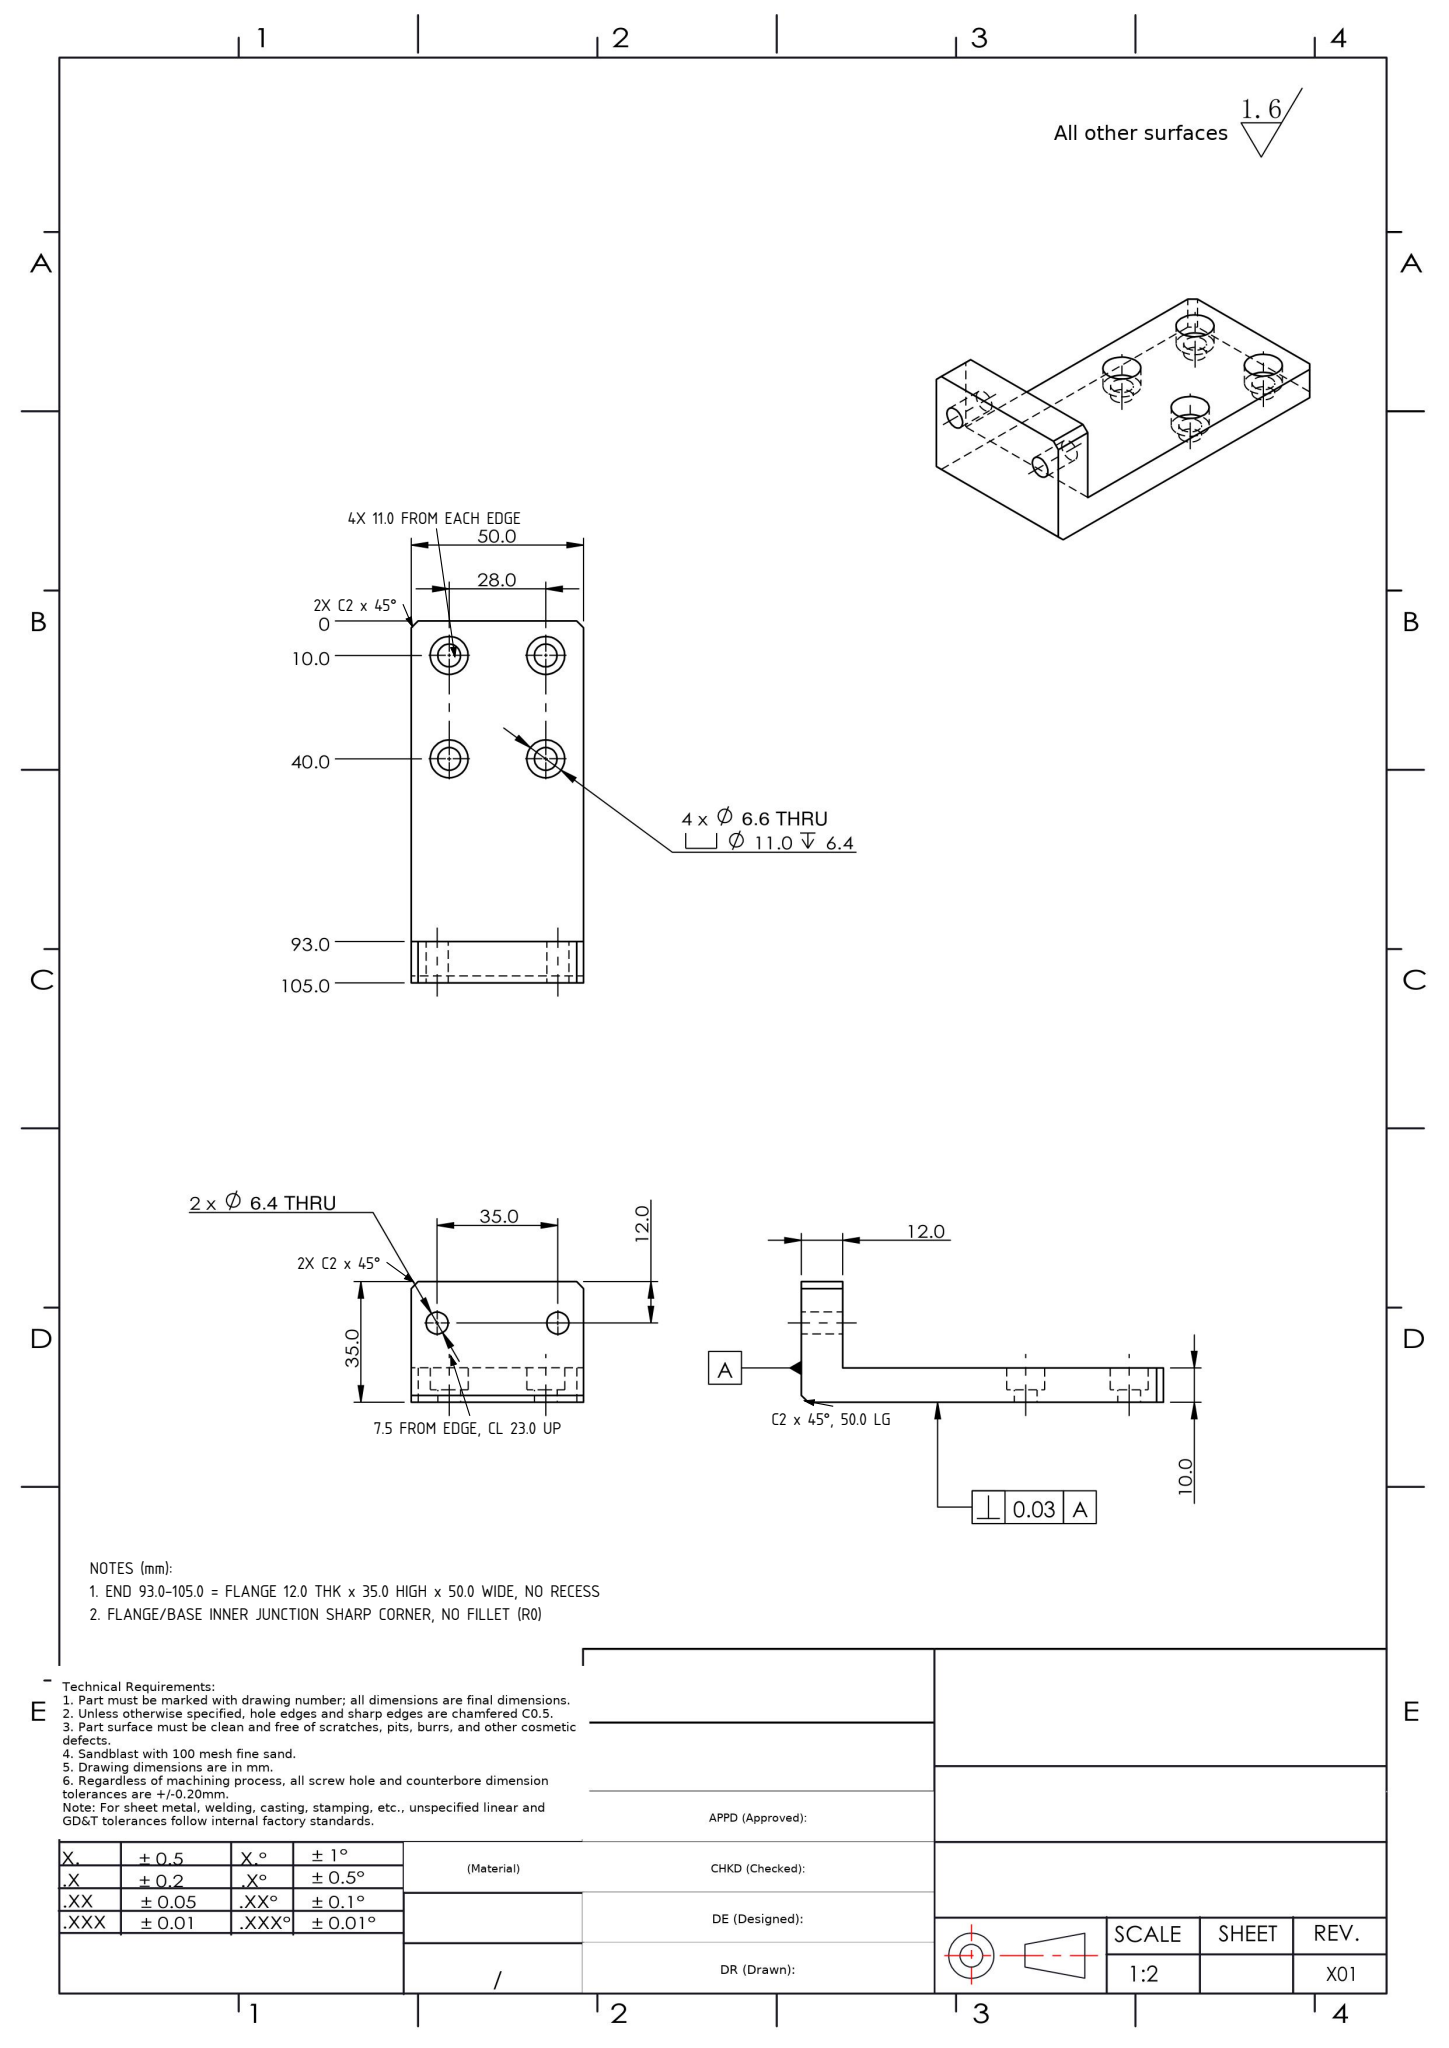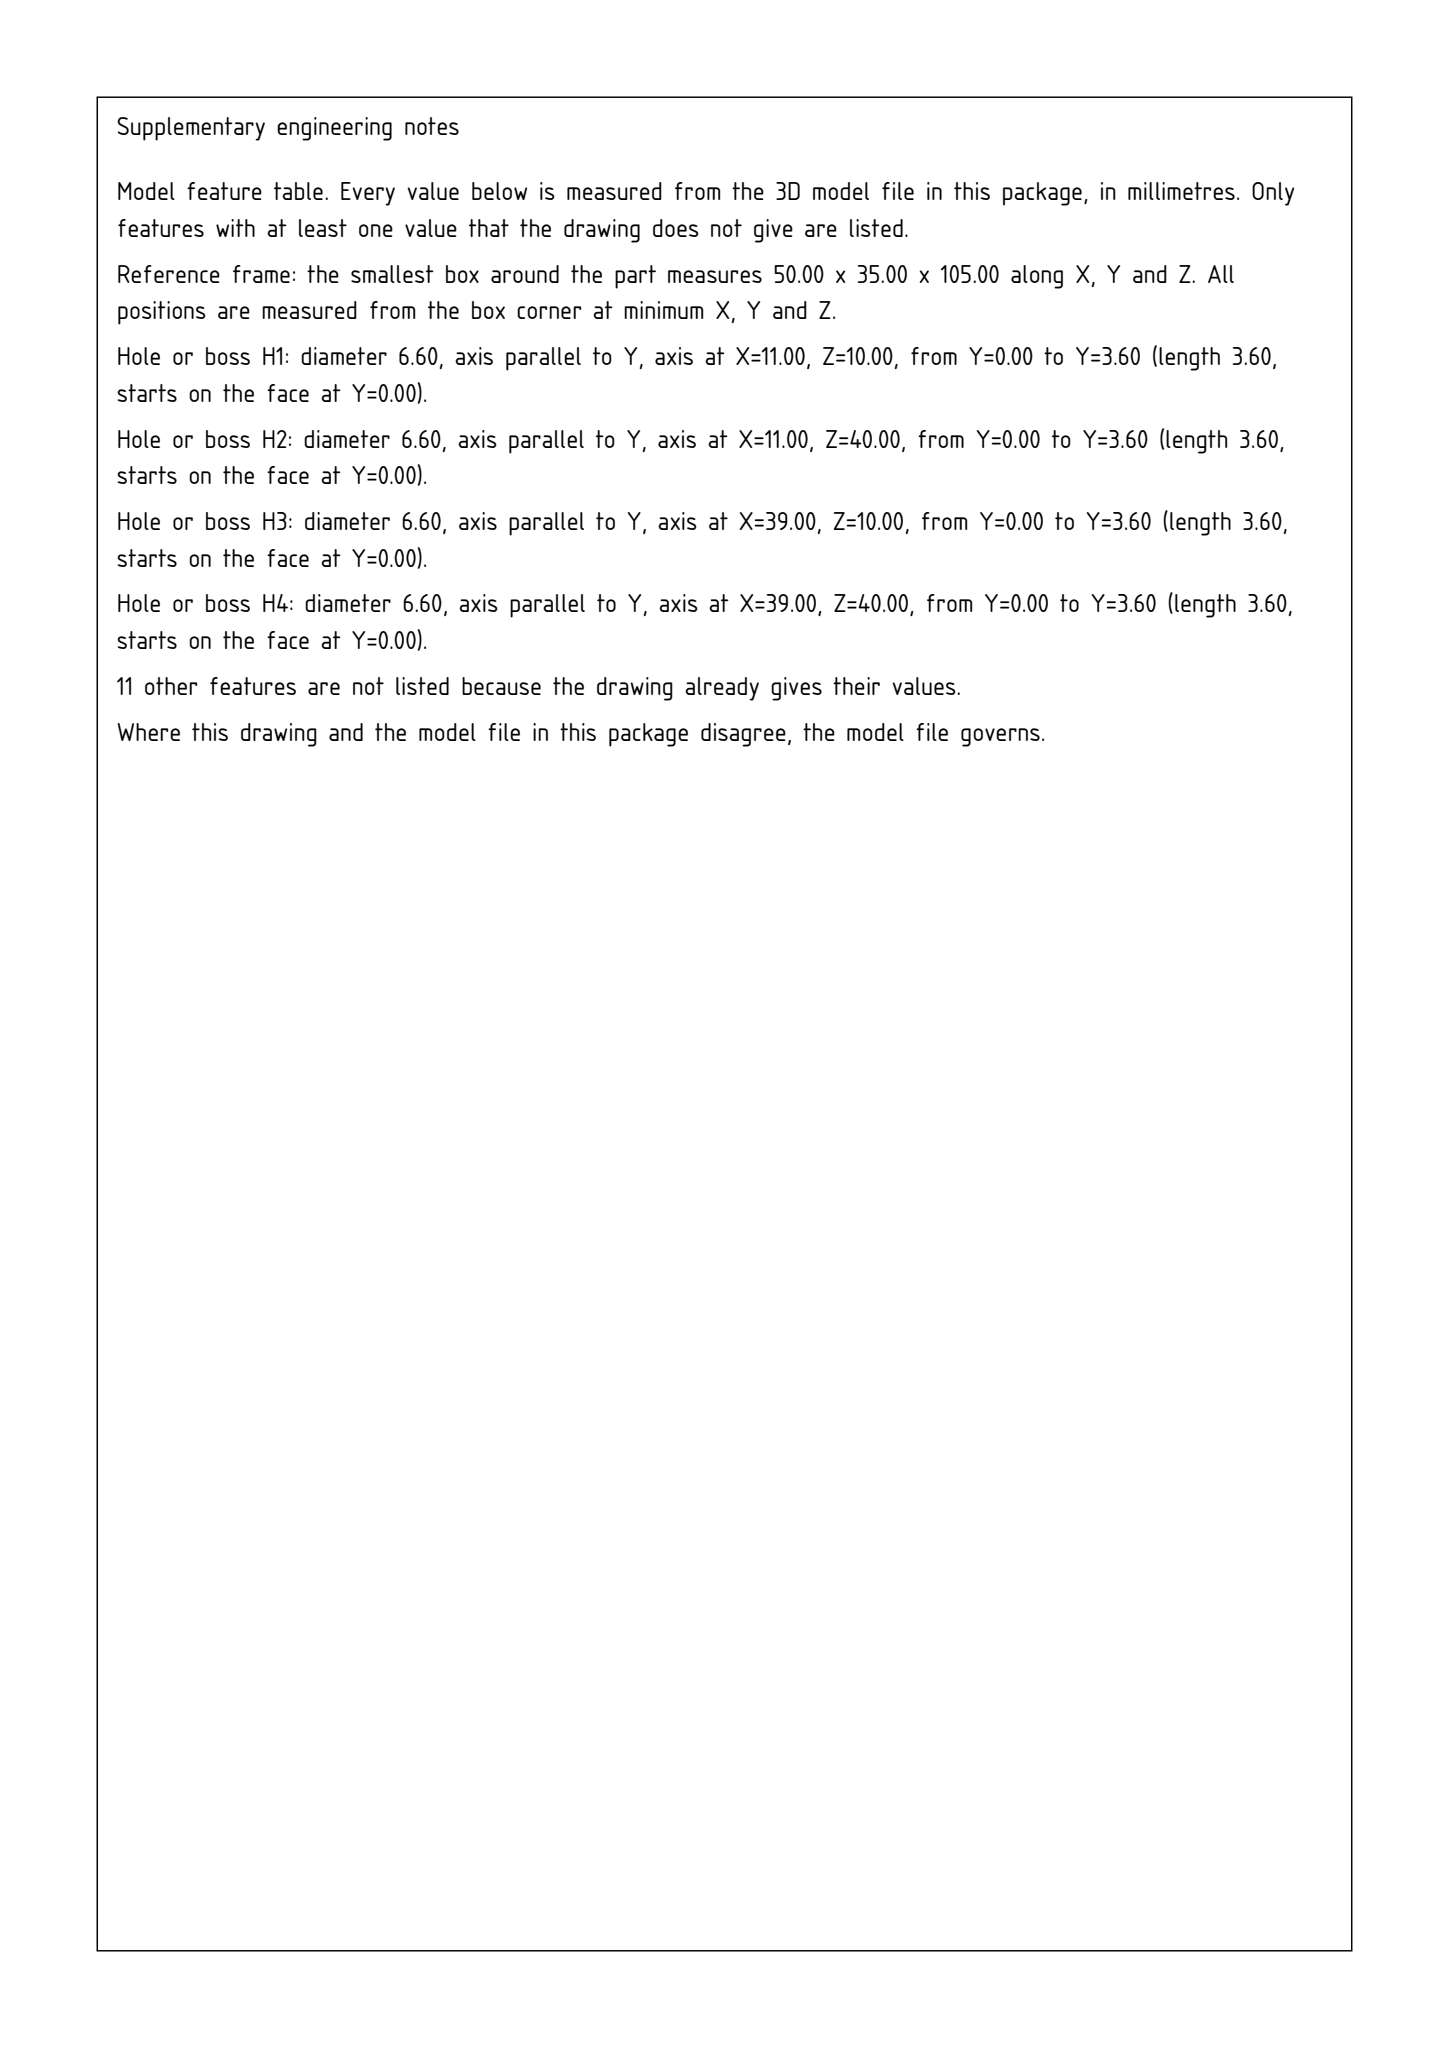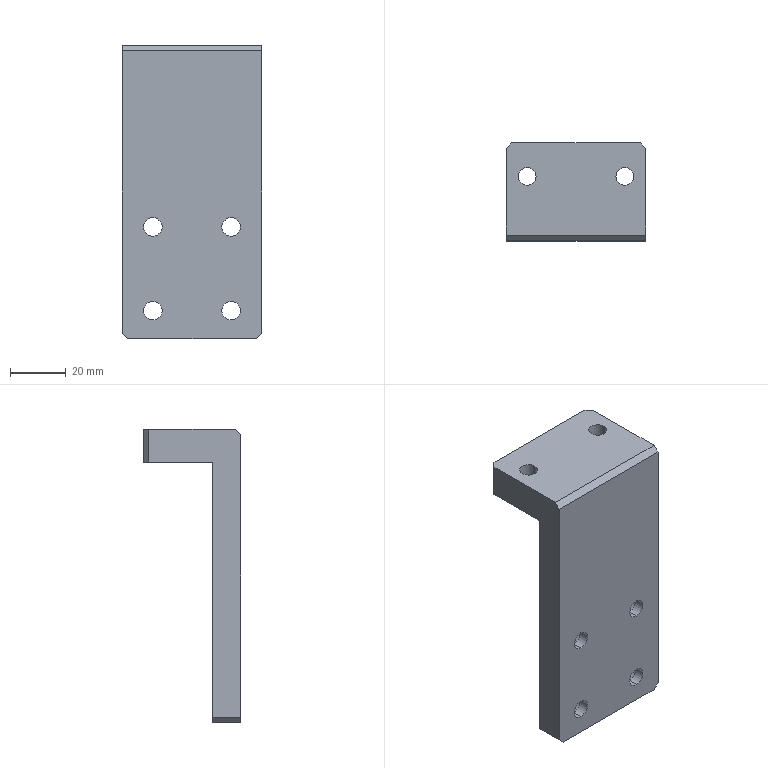Part | SolidWorks | mm | 1 solid | 37 faces | box 50 x 35 x 105 mm | volume 63614 mm3 | cylinder 20 | plane 17 | commonest cylinder face diameters 11 x8 6.6 x8 6.4 x4
Drawing notes:
END 93.0-105.0 = FLANGE 12.0 THK x 35.0 HIGH x 50.0 WIDE, NO RECESS | from the solid: Planes z=93 & z=105 (12 apart), y=0 to 35, x=0 to 50; base only y=0-10
FLANGE/BASE INNER JUNCTION SHARP CORNER, NO FILLET (R0) | from the solid: "fillet_radii": [] - no radii present in model
4 x Ø6.6 CBORE HOLES SYM ABOUT 50.0 WIDTH CL, 11.0 FROM EACH EDGE | from the solid: Ø6.6/Ø11.0 cyl axes at x=11.0 and x=39.0, x-planes at 0 and 50.0
2 x Ø6.4 THRU SYM ABOUT 50.0 WIDTH CL, 7.5 FROM EACH EDGE, CL 23.0 UP FROM BASE BTM | from the solid: Ø6.4 cyl axes at (x=7.5,y=23) and (x=42.5,y=23), length 12; x-planes 0 and 50.0
C2 x 45 ON FRONT FACE EDGE AT 105.0 END, 50.0 LG | from the solid: inclined plane 45/45 to Y,Z at bbox_from [0,0,103], size [50,2,2] (y=0 / z=105 edge)
2 x C2 x 45 ON FLANGE OUTER CORNERS AT 35.0, 12.0 LG | from the solid: two inclined planes 45/45 to X,Y at [0,33,93] and [48,33,93], size [2,2,12]
2 x C2 x 45 ON BOTH CORNERS AT 0 END OF PLATE, 10.0 LG | from the solid: two inclined planes 45/45 to X,Z at [0,0,0] and [48,0,0], size [2,10,2]
build123d program:
from build123d import *

# Parameters (mm, degrees)
SKETCH1_W                                       = 50
SKETCH1_H                                       = 105
BOSS_EXTRUDE1_DEPTH                             = 10
SKETCH2_W                                       = 50
SKETCH2_H                                       = 12
BOSS_EXTRUDE2_DEPTH                             = 25
CHAMFER1_SIZE                                   = 2
M6_CLEARANCE_SLOT1_D                            = 6.4
M6_HEX_SOCKET_HEAD_CAP_SCREW_CBORE1_D           = 6.6
M6_HEX_SOCKET_HEAD_CAP_SCREW_CBORE1_CBORE_D     = 11
M6_HEX_SOCKET_HEAD_CAP_SCREW_CBORE1_CBORE_DEPTH = 6.4
LPATTERN1_COUNT                                 = 2
LPATTERN1_PITCH                                 = 30


with BuildPart() as part:
    # Sketch1 → Boss-Extrude1 (new body)
    with BuildSketch(Plane(origin=(0, 0, 0), x_dir=(1, 0, 0), z_dir=(0, 1, 0))):
        Rectangle(SKETCH1_W, SKETCH1_H)
    extrude(amount=BOSS_EXTRUDE1_DEPTH)

    # Sketch2 → Boss-Extrude2 (add)
    with BuildSketch(Plane(origin=(0, 10, 0), x_dir=(1, 0, 0), z_dir=(0, 1, 0))):
        with Locations((0, -46.5)):
            Rectangle(SKETCH2_W, SKETCH2_H)
    extrude(amount=BOSS_EXTRUDE2_DEPTH)

    # Chamfer1
    chamfer1_edges = [part.edges().sort_by_distance(p)[0] for p in [
        (0, 0, 52.5),
        (-25, 35, 46.5),
        (25, 35, 46.5),
        (25, 5, -52.5),
        (-25, 5, -52.5),
    ]]
    chamfer(chamfer1_edges, length=CHAMFER1_SIZE)

    # M6 Clearance Slot1 (through all)
    with Locations(Plane(origin=(0, 0, 40.5), x_dir=(-1, 0, 0), z_dir=(0, 0, -1))):
        with Locations((17.5, 23), (-17.5, 23)):
            Hole(M6_CLEARANCE_SLOT1_D / 2)

    # M6 Hex Socket Head Cap Screw CBORE1 (through all)
    with Locations(Plane(origin=(0, 10, 0), x_dir=(1, 0, 0), z_dir=(0, 1, 0))):
        with Locations((-14, 42.5), (14, 42.5)):
            m6_hex_socket_head_cap_screw_cbore1 = CounterBoreHole(M6_HEX_SOCKET_HEAD_CAP_SCREW_CBORE1_D / 2, M6_HEX_SOCKET_HEAD_CAP_SCREW_CBORE1_CBORE_D / 2, M6_HEX_SOCKET_HEAD_CAP_SCREW_CBORE1_CBORE_DEPTH)

    # LPattern1: M6 Hex Socket Head Cap Screw CBORE1 ×2
    with Locations(*[(0, 0, i * LPATTERN1_PITCH) for i in range(1, LPATTERN1_COUNT)]):
        add(m6_hex_socket_head_cap_screw_cbore1, mode=Mode.SUBTRACT)


solid = part.part